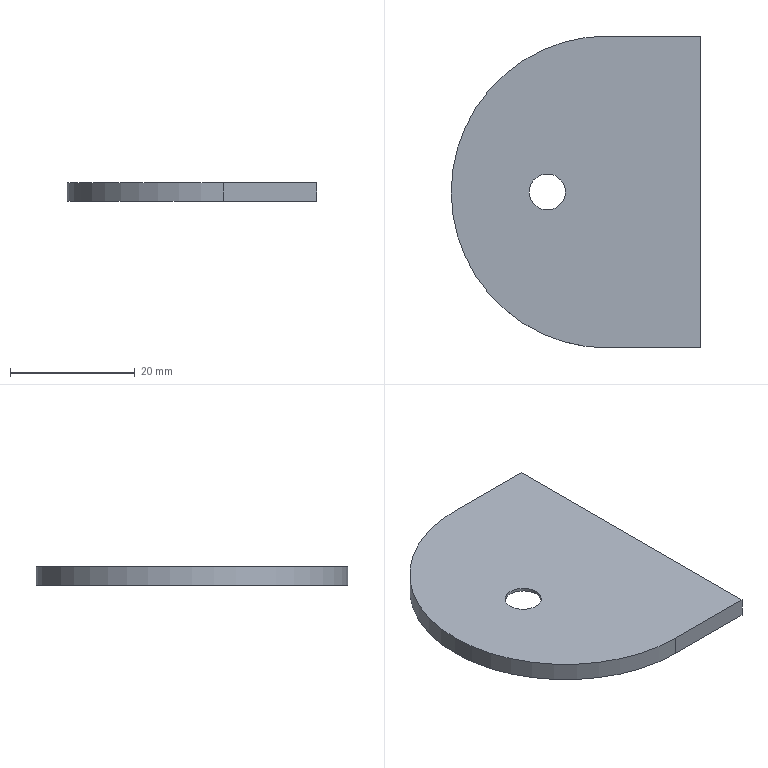Component | NX | HOUSING_COVER | 1 solid | 12 faces | box 40 x 50 x 3 mm | volume 1049 mm3 | plane 9 | cylinder 3 | commonest cylinder face diameters 50 x1 49 x1 5.8 x1
STEP:
#1=CARTESIAN_POINT('',(0.,0.,0.));
#2=DIRECTION('',(0.,0.,1.));
#3=DIRECTION('',(1.,0.,0.));
#4=AXIS2_PLACEMENT_3D('',#1,#2,#3);
#5=CARTESIAN_POINT('',(40.11,76.025,23.712));
#6=VERTEX_POINT('',#5);
#7=CARTESIAN_POINT('',(40.11,26.025,23.712));
#8=VERTEX_POINT('',#7);
#9=CARTESIAN_POINT('',(40.11,51.025,23.712));
#10=DIRECTION('',(0.,0.,1.));
#11=DIRECTION('',(1.,0.,0.));
#12=AXIS2_PLACEMENT_3D('',#9,#10,#11);
#13=CIRCLE('',#12,25.);
#14=CARTESIAN_POINT('',(40.11,51.025,20.712));
#15=DIRECTION('',(0.,0.,1.));
#16=DIRECTION('',(1.,0.,0.));
#17=AXIS2_PLACEMENT_3D('',#14,#15,#16);
#18=CYLINDRICAL_SURFACE('',#17,25.);
#19=CARTESIAN_POINT('',(0.,3.));
#20=DIRECTION('',(1.,0.));
#21=VECTOR('',#20,1.);
#22=LINE('',#19,#21);
#23=(GEOMETRIC_REPRESENTATION_CONTEXT(2)PARAMETRIC_REPRESENTATION_CONTEXT()REPRESENTATION_CONTEXT('',''));
#24=DEFINITIONAL_REPRESENTATION('',(#22),#23);
#25=PCURVE('',#18,#24);
#26=CARTESIAN_POINT('',(40.11,51.025,23.712));
#27=DIRECTION('',(0.,0.,1.));
#28=DIRECTION('',(1.,0.,0.));
#29=AXIS2_PLACEMENT_3D('',#26,#27,#28);
#30=PLANE('',#29);
#31=CARTESIAN_POINT('',(0.,0.));
#32=DIRECTION('',(1.,0.));
#33=AXIS2_PLACEMENT_2D('',#31,#32);
#34=CIRCLE('',#33,25.);
#35=(GEOMETRIC_REPRESENTATION_CONTEXT(2)PARAMETRIC_REPRESENTATION_CONTEXT()REPRESENTATION_CONTEXT('',''));
#36=DEFINITIONAL_REPRESENTATION('',(#34),#35);
#37=PCURVE('',#30,#36);
#38=SURFACE_CURVE('',#13,(#25,#37),.PCURVE_S1.);
#39=EDGE_CURVE('',#6,#8,#38,.T.);
#40=ORIENTED_EDGE('',*,*,#39,.F.);
#41=CARTESIAN_POINT('',(40.11,76.025,20.712));
#42=VERTEX_POINT('',#41);
#43=CARTESIAN_POINT('',(40.11,76.025,20.712));
#44=DIRECTION('',(0.,0.,1.));
#45=VECTOR('',#44,1.);
#46=LINE('',#43,#45);
#47=CARTESIAN_POINT('',(1.571,0.));
#48=DIRECTION('',(0.,1.));
#49=VECTOR('',#48,1.);
#50=LINE('',#47,#49);
#51=(GEOMETRIC_REPRESENTATION_CONTEXT(2)PARAMETRIC_REPRESENTATION_CONTEXT()REPRESENTATION_CONTEXT('',''));
#52=DEFINITIONAL_REPRESENTATION('',(#50),#51);
#53=PCURVE('',#18,#52);
#54=CARTESIAN_POINT('',(55.11,76.025,20.712));
#55=DIRECTION('',(0.,1.,0.));
#56=DIRECTION('',(0.,0.,1.));
#57=AXIS2_PLACEMENT_3D('',#54,#55,#56);
#58=PLANE('',#57);
#59=CARTESIAN_POINT('',(0.,-15.));
#60=DIRECTION('',(1.,0.));
#61=VECTOR('',#60,1.);
#62=LINE('',#59,#61);
#63=(GEOMETRIC_REPRESENTATION_CONTEXT(2)PARAMETRIC_REPRESENTATION_CONTEXT()REPRESENTATION_CONTEXT('',''));
#64=DEFINITIONAL_REPRESENTATION('',(#62),#63);
#65=PCURVE('',#58,#64);
#66=SURFACE_CURVE('',#46,(#53,#65),.PCURVE_S1.);
#67=EDGE_CURVE('',#42,#6,#66,.T.);
#68=ORIENTED_EDGE('',*,*,#67,.F.);
#69=CARTESIAN_POINT('',(40.11,26.025,20.712));
#70=VERTEX_POINT('',#69);
#71=CARTESIAN_POINT('',(40.11,51.025,20.712));
#72=DIRECTION('',(0.,0.,1.));
#73=DIRECTION('',(1.,0.,0.));
#74=AXIS2_PLACEMENT_3D('',#71,#72,#73);
#75=CIRCLE('',#74,25.);
#76=CARTESIAN_POINT('',(0.,0.));
#77=DIRECTION('',(1.,0.));
#78=VECTOR('',#77,1.);
#79=LINE('',#76,#78);
#80=(GEOMETRIC_REPRESENTATION_CONTEXT(2)PARAMETRIC_REPRESENTATION_CONTEXT()REPRESENTATION_CONTEXT('',''));
#81=DEFINITIONAL_REPRESENTATION('',(#79),#80);
#82=PCURVE('',#18,#81);
#83=CARTESIAN_POINT('',(40.11,51.025,20.712));
#84=DIRECTION('',(0.,0.,1.));
#85=DIRECTION('',(1.,0.,0.));
#86=AXIS2_PLACEMENT_3D('',#83,#84,#85);
#87=PLANE('',#86);
#88=CARTESIAN_POINT('',(0.,0.));
#89=DIRECTION('',(1.,0.));
#90=AXIS2_PLACEMENT_2D('',#88,#89);
#91=CIRCLE('',#90,25.);
#92=(GEOMETRIC_REPRESENTATION_CONTEXT(2)PARAMETRIC_REPRESENTATION_CONTEXT()REPRESENTATION_CONTEXT('',''));
#93=DEFINITIONAL_REPRESENTATION('',(#91),#92);
#94=PCURVE('',#87,#93);
#95=SURFACE_CURVE('',#75,(#82,#94),.PCURVE_S1.);
#96=EDGE_CURVE('',#42,#70,#95,.T.);
#97=ORIENTED_EDGE('',*,*,#96,.T.);
#98=CARTESIAN_POINT('',(40.11,26.025,20.712));
#99=DIRECTION('',(0.,0.,1.));
#100=VECTOR('',#99,1.);
#101=LINE('',#98,#100);
#102=CARTESIAN_POINT('',(4.712,0.));
#103=DIRECTION('',(0.,1.));
#104=VECTOR('',#103,1.);
#105=LINE('',#102,#104);
#106=(GEOMETRIC_REPRESENTATION_CONTEXT(2)PARAMETRIC_REPRESENTATION_CONTEXT()REPRESENTATION_CONTEXT('',''));
#107=DEFINITIONAL_REPRESENTATION('',(#105),#106);
#108=PCURVE('',#18,#107);
#109=CARTESIAN_POINT('',(40.11,26.025,20.712));
#110=DIRECTION('',(0.,-1.,0.));
#111=DIRECTION('',(0.,0.,-1.));
#112=AXIS2_PLACEMENT_3D('',#109,#110,#111);
#113=PLANE('',#112);
#114=CARTESIAN_POINT('',(0.,0.));
#115=DIRECTION('',(-1.,0.));
#116=VECTOR('',#115,1.);
#117=LINE('',#114,#116);
#118=(GEOMETRIC_REPRESENTATION_CONTEXT(2)PARAMETRIC_REPRESENTATION_CONTEXT()REPRESENTATION_CONTEXT('',''));
#119=DEFINITIONAL_REPRESENTATION('',(#117),#118);
#120=PCURVE('',#113,#119);
#121=SURFACE_CURVE('',#101,(#108,#120),.PCURVE_S1.);
#122=EDGE_CURVE('',#70,#8,#121,.T.);
#123=ORIENTED_EDGE('',*,*,#122,.T.);
#124=EDGE_LOOP('',(#40,#68,#97,#123));
#125=FACE_BOUND('',#124,.T.);
#126=ADVANCED_FACE('',(#125),#18,.T.);
#127=CARTESIAN_POINT('',(55.11,26.025,23.712));
#128=VERTEX_POINT('',#127);
#129=CARTESIAN_POINT('',(40.11,26.025,23.712));
#130=DIRECTION('',(1.,0.,0.));
#131=VECTOR('',#130,1.);
#132=LINE('',#129,#131);
#133=CARTESIAN_POINT('',(-3.,0.));
#134=DIRECTION('',(0.,1.));
#135=VECTOR('',#134,1.);
#136=LINE('',#133,#135);
#137=(GEOMETRIC_REPRESENTATION_CONTEXT(2)PARAMETRIC_REPRESENTATION_CONTEXT()REPRESENTATION_CONTEXT('',''));
#138=DEFINITIONAL_REPRESENTATION('',(#136),#137);
#139=PCURVE('',#113,#138);
#140=CARTESIAN_POINT('',(0.,-25.));
#141=DIRECTION('',(1.,0.));
#142=VECTOR('',#141,1.);
#143=LINE('',#140,#142);
#144=(GEOMETRIC_REPRESENTATION_CONTEXT(2)PARAMETRIC_REPRESENTATION_CONTEXT()REPRESENTATION_CONTEXT('',''));
#145=DEFINITIONAL_REPRESENTATION('',(#143),#144);
#146=PCURVE('',#30,#145);
#147=SURFACE_CURVE('',#132,(#139,#146),.PCURVE_S1.);
#148=EDGE_CURVE('',#8,#128,#147,.T.);
#149=ORIENTED_EDGE('',*,*,#148,.F.);
#150=ORIENTED_EDGE('',*,*,#122,.F.);
#151=CARTESIAN_POINT('',(55.11,26.025,20.712));
#152=VERTEX_POINT('',#151);
#153=CARTESIAN_POINT('',(40.11,26.025,20.712));
#154=DIRECTION('',(1.,0.,0.));
#155=VECTOR('',#154,1.);
#156=LINE('',#153,#155);
#157=CARTESIAN_POINT('',(0.,0.));
#158=DIRECTION('',(0.,1.));
#159=VECTOR('',#158,1.);
#160=LINE('',#157,#159);
#161=(GEOMETRIC_REPRESENTATION_CONTEXT(2)PARAMETRIC_REPRESENTATION_CONTEXT()REPRESENTATION_CONTEXT('',''));
#162=DEFINITIONAL_REPRESENTATION('',(#160),#161);
#163=PCURVE('',#113,#162);
#164=CARTESIAN_POINT('',(0.,-25.));
#165=DIRECTION('',(1.,0.));
#166=VECTOR('',#165,1.);
#167=LINE('',#164,#166);
#168=(GEOMETRIC_REPRESENTATION_CONTEXT(2)PARAMETRIC_REPRESENTATION_CONTEXT()REPRESENTATION_CONTEXT('',''));
#169=DEFINITIONAL_REPRESENTATION('',(#167),#168);
#170=PCURVE('',#87,#169);
#171=SURFACE_CURVE('',#156,(#163,#170),.PCURVE_S1.);
#172=EDGE_CURVE('',#70,#152,#171,.T.);
#173=ORIENTED_EDGE('',*,*,#172,.T.);
#174=CARTESIAN_POINT('',(55.11,26.025,20.712));
#175=DIRECTION('',(0.,0.,1.));
#176=VECTOR('',#175,1.);
#177=LINE('',#174,#176);
#178=CARTESIAN_POINT('',(0.,15.));
#179=DIRECTION('',(-1.,0.));
#180=VECTOR('',#179,1.);
#181=LINE('',#178,#180);
#182=(GEOMETRIC_REPRESENTATION_CONTEXT(2)PARAMETRIC_REPRESENTATION_CONTEXT()REPRESENTATION_CONTEXT('',''));
#183=DEFINITIONAL_REPRESENTATION('',(#181),#182);
#184=PCURVE('',#113,#183);
#185=CARTESIAN_POINT('',(55.11,26.025,20.712));
#186=DIRECTION('',(1.,0.,0.));
#187=DIRECTION('',(-0.,1.,0.));
#188=AXIS2_PLACEMENT_3D('',#185,#186,#187);
#189=PLANE('',#188);
#190=CARTESIAN_POINT('',(0.,0.));
#191=DIRECTION('',(0.,1.));
#192=VECTOR('',#191,1.);
#193=LINE('',#190,#192);
#194=(GEOMETRIC_REPRESENTATION_CONTEXT(2)PARAMETRIC_REPRESENTATION_CONTEXT()REPRESENTATION_CONTEXT('',''));
#195=DEFINITIONAL_REPRESENTATION('',(#193),#194);
#196=PCURVE('',#189,#195);
#197=SURFACE_CURVE('',#177,(#184,#196),.PCURVE_S1.);
#198=EDGE_CURVE('',#152,#128,#197,.T.);
#199=ORIENTED_EDGE('',*,*,#198,.T.);
#200=EDGE_LOOP('',(#149,#150,#173,#199));
#201=FACE_BOUND('',#200,.T.);
#202=ADVANCED_FACE('',(#201),#113,.T.);
#203=CARTESIAN_POINT('',(55.11,76.025,23.712));
#204=VERTEX_POINT('',#203);
#205=CARTESIAN_POINT('',(55.11,26.025,23.712));
#206=DIRECTION('',(-0.,1.,0.));
#207=VECTOR('',#206,1.);
#208=LINE('',#205,#207);
#209=CARTESIAN_POINT('',(0.,3.));
#210=DIRECTION('',(1.,0.));
#211=VECTOR('',#210,1.);
#212=LINE('',#209,#211);
#213=(GEOMETRIC_REPRESENTATION_CONTEXT(2)PARAMETRIC_REPRESENTATION_CONTEXT()REPRESENTATION_CONTEXT('',''));
#214=DEFINITIONAL_REPRESENTATION('',(#212),#213);
#215=PCURVE('',#189,#214);
#216=CARTESIAN_POINT('',(15.,-25.));
#217=DIRECTION('',(-0.,1.));
#218=VECTOR('',#217,1.);
#219=LINE('',#216,#218);
#220=(GEOMETRIC_REPRESENTATION_CONTEXT(2)PARAMETRIC_REPRESENTATION_CONTEXT()REPRESENTATION_CONTEXT('',''));
#221=DEFINITIONAL_REPRESENTATION('',(#219),#220);
#222=PCURVE('',#30,#221);
#223=SURFACE_CURVE('',#208,(#215,#222),.PCURVE_S1.);
#224=EDGE_CURVE('',#128,#204,#223,.T.);
#225=ORIENTED_EDGE('',*,*,#224,.F.);
#226=ORIENTED_EDGE('',*,*,#198,.F.);
#227=CARTESIAN_POINT('',(55.11,76.025,20.712));
#228=VERTEX_POINT('',#227);
#229=CARTESIAN_POINT('',(55.11,26.025,20.712));
#230=DIRECTION('',(-0.,1.,0.));
#231=VECTOR('',#230,1.);
#232=LINE('',#229,#231);
#233=CARTESIAN_POINT('',(0.,0.));
#234=DIRECTION('',(1.,0.));
#235=VECTOR('',#234,1.);
#236=LINE('',#233,#235);
#237=(GEOMETRIC_REPRESENTATION_CONTEXT(2)PARAMETRIC_REPRESENTATION_CONTEXT()REPRESENTATION_CONTEXT('',''));
#238=DEFINITIONAL_REPRESENTATION('',(#236),#237);
#239=PCURVE('',#189,#238);
#240=CARTESIAN_POINT('',(15.,-25.));
#241=DIRECTION('',(-0.,1.));
#242=VECTOR('',#241,1.);
#243=LINE('',#240,#242);
#244=(GEOMETRIC_REPRESENTATION_CONTEXT(2)PARAMETRIC_REPRESENTATION_CONTEXT()REPRESENTATION_CONTEXT('',''));
#245=DEFINITIONAL_REPRESENTATION('',(#243),#244);
#246=PCURVE('',#87,#245);
#247=SURFACE_CURVE('',#232,(#239,#246),.PCURVE_S1.);
#248=EDGE_CURVE('',#152,#228,#247,.T.);
#249=ORIENTED_EDGE('',*,*,#248,.T.);
#250=CARTESIAN_POINT('',(55.11,76.025,20.712));
#251=DIRECTION('',(0.,0.,1.));
#252=VECTOR('',#251,1.);
#253=LINE('',#250,#252);
#254=CARTESIAN_POINT('',(50.,0.));
#255=DIRECTION('',(0.,1.));
#256=VECTOR('',#255,1.);
#257=LINE('',#254,#256);
#258=(GEOMETRIC_REPRESENTATION_CONTEXT(2)PARAMETRIC_REPRESENTATION_CONTEXT()REPRESENTATION_CONTEXT('',''));
#259=DEFINITIONAL_REPRESENTATION('',(#257),#258);
#260=PCURVE('',#189,#259);
#261=CARTESIAN_POINT('',(0.,0.));
#262=DIRECTION('',(1.,0.));
#263=VECTOR('',#262,1.);
#264=LINE('',#261,#263);
#265=(GEOMETRIC_REPRESENTATION_CONTEXT(2)PARAMETRIC_REPRESENTATION_CONTEXT()REPRESENTATION_CONTEXT('',''));
#266=DEFINITIONAL_REPRESENTATION('',(#264),#265);
#267=PCURVE('',#58,#266);
#268=SURFACE_CURVE('',#253,(#260,#267),.PCURVE_S1.);
#269=EDGE_CURVE('',#228,#204,#268,.T.);
#270=ORIENTED_EDGE('',*,*,#269,.T.);
#271=EDGE_LOOP('',(#225,#226,#249,#270));
#272=FACE_BOUND('',#271,.T.);
#273=ADVANCED_FACE('',(#272),#189,.T.);
#274=CARTESIAN_POINT('',(55.11,76.025,23.712));
#275=DIRECTION('',(-1.,0.,0.));
#276=VECTOR('',#275,1.);
#277=LINE('',#274,#276);
#278=CARTESIAN_POINT('',(3.,0.));
#279=DIRECTION('',(0.,-1.));
#280=VECTOR('',#279,1.);
#281=LINE('',#278,#280);
#282=(GEOMETRIC_REPRESENTATION_CONTEXT(2)PARAMETRIC_REPRESENTATION_CONTEXT()REPRESENTATION_CONTEXT('',''));
#283=DEFINITIONAL_REPRESENTATION('',(#281),#282);
#284=PCURVE('',#58,#283);
#285=CARTESIAN_POINT('',(15.,25.));
#286=DIRECTION('',(-1.,0.));
#287=VECTOR('',#286,1.);
#288=LINE('',#285,#287);
#289=(GEOMETRIC_REPRESENTATION_CONTEXT(2)PARAMETRIC_REPRESENTATION_CONTEXT()REPRESENTATION_CONTEXT('',''));
#290=DEFINITIONAL_REPRESENTATION('',(#288),#289);
#291=PCURVE('',#30,#290);
#292=SURFACE_CURVE('',#277,(#284,#291),.PCURVE_S1.);
#293=EDGE_CURVE('',#204,#6,#292,.T.);
#294=ORIENTED_EDGE('',*,*,#293,.F.);
#295=ORIENTED_EDGE('',*,*,#269,.F.);
#296=CARTESIAN_POINT('',(55.11,76.025,20.712));
#297=DIRECTION('',(-1.,0.,0.));
#298=VECTOR('',#297,1.);
#299=LINE('',#296,#298);
#300=CARTESIAN_POINT('',(0.,0.));
#301=DIRECTION('',(0.,-1.));
#302=VECTOR('',#301,1.);
#303=LINE('',#300,#302);
#304=(GEOMETRIC_REPRESENTATION_CONTEXT(2)PARAMETRIC_REPRESENTATION_CONTEXT()REPRESENTATION_CONTEXT('',''));
#305=DEFINITIONAL_REPRESENTATION('',(#303),#304);
#306=PCURVE('',#58,#305);
#307=CARTESIAN_POINT('',(15.,25.));
#308=DIRECTION('',(-1.,0.));
#309=VECTOR('',#308,1.);
#310=LINE('',#307,#309);
#311=(GEOMETRIC_REPRESENTATION_CONTEXT(2)PARAMETRIC_REPRESENTATION_CONTEXT()REPRESENTATION_CONTEXT('',''));
#312=DEFINITIONAL_REPRESENTATION('',(#310),#311);
#313=PCURVE('',#87,#312);
#314=SURFACE_CURVE('',#299,(#306,#313),.PCURVE_S1.);
#315=EDGE_CURVE('',#228,#42,#314,.T.);
#316=ORIENTED_EDGE('',*,*,#315,.T.);
#317=ORIENTED_EDGE('',*,*,#67,.T.);
#318=EDGE_LOOP('',(#294,#295,#316,#317));
#319=FACE_BOUND('',#318,.T.);
#320=ADVANCED_FACE('',(#319),#58,.T.);
#321=CARTESIAN_POINT('',(54.61,75.525,20.712));
#322=VERTEX_POINT('',#321);
#323=CARTESIAN_POINT('',(40.11,75.525,20.712));
#324=VERTEX_POINT('',#323);
#325=CARTESIAN_POINT('',(40.11,75.525,20.712));
#326=DIRECTION('',(-1.,0.,0.));
#327=VECTOR('',#326,1.);
#328=LINE('',#325,#327);
#329=CARTESIAN_POINT('',(0.,24.5));
#330=DIRECTION('',(-1.,0.));
#331=VECTOR('',#330,1.);
#332=LINE('',#329,#331);
#333=(GEOMETRIC_REPRESENTATION_CONTEXT(2)PARAMETRIC_REPRESENTATION_CONTEXT()REPRESENTATION_CONTEXT('',''));
#334=DEFINITIONAL_REPRESENTATION('',(#332),#333);
#335=PCURVE('',#87,#334);
#336=CARTESIAN_POINT('',(55.11,75.525,20.712));
#337=DIRECTION('',(0.,1.,0.));
#338=DIRECTION('',(0.,0.,1.));
#339=AXIS2_PLACEMENT_3D('',#336,#337,#338);
#340=PLANE('',#339);
#341=CARTESIAN_POINT('',(0.,-15.));
#342=DIRECTION('',(0.,-1.));
#343=VECTOR('',#342,1.);
#344=LINE('',#341,#343);
#345=(GEOMETRIC_REPRESENTATION_CONTEXT(2)PARAMETRIC_REPRESENTATION_CONTEXT()REPRESENTATION_CONTEXT('',''));
#346=DEFINITIONAL_REPRESENTATION('',(#344),#345);
#347=PCURVE('',#340,#346);
#348=SURFACE_CURVE('',#328,(#335,#347),.PCURVE_S1.);
#349=EDGE_CURVE('',#322,#324,#348,.T.);
#350=ORIENTED_EDGE('',*,*,#349,.T.);
#351=CARTESIAN_POINT('',(40.11,26.525,20.712));
#352=VERTEX_POINT('',#351);
#353=CARTESIAN_POINT('',(40.11,51.025,20.712));
#354=DIRECTION('',(0.,0.,1.));
#355=DIRECTION('',(1.,0.,0.));
#356=AXIS2_PLACEMENT_3D('',#353,#354,#355);
#357=CIRCLE('',#356,24.5);
#358=CARTESIAN_POINT('',(0.,0.));
#359=DIRECTION('',(1.,0.));
#360=AXIS2_PLACEMENT_2D('',#358,#359);
#361=CIRCLE('',#360,24.5);
#362=(GEOMETRIC_REPRESENTATION_CONTEXT(2)PARAMETRIC_REPRESENTATION_CONTEXT()REPRESENTATION_CONTEXT('',''));
#363=DEFINITIONAL_REPRESENTATION('',(#361),#362);
#364=PCURVE('',#87,#363);
#365=CARTESIAN_POINT('',(40.11,51.025,20.712));
#366=DIRECTION('',(0.,0.,1.));
#367=DIRECTION('',(1.,0.,0.));
#368=AXIS2_PLACEMENT_3D('',#365,#366,#367);
#369=CYLINDRICAL_SURFACE('',#368,24.5);
#370=CARTESIAN_POINT('',(0.,0.));
#371=DIRECTION('',(1.,0.));
#372=VECTOR('',#371,1.);
#373=LINE('',#370,#372);
#374=(GEOMETRIC_REPRESENTATION_CONTEXT(2)PARAMETRIC_REPRESENTATION_CONTEXT()REPRESENTATION_CONTEXT('',''));
#375=DEFINITIONAL_REPRESENTATION('',(#373),#374);
#376=PCURVE('',#369,#375);
#377=SURFACE_CURVE('',#357,(#364,#376),.PCURVE_S1.);
#378=EDGE_CURVE('',#324,#352,#377,.T.);
#379=ORIENTED_EDGE('',*,*,#378,.T.);
#380=CARTESIAN_POINT('',(54.61,26.525,20.712));
#381=VERTEX_POINT('',#380);
#382=CARTESIAN_POINT('',(40.11,26.525,20.712));
#383=DIRECTION('',(1.,0.,0.));
#384=VECTOR('',#383,1.);
#385=LINE('',#382,#384);
#386=CARTESIAN_POINT('',(0.,-24.5));
#387=DIRECTION('',(1.,0.));
#388=VECTOR('',#387,1.);
#389=LINE('',#386,#388);
#390=(GEOMETRIC_REPRESENTATION_CONTEXT(2)PARAMETRIC_REPRESENTATION_CONTEXT()REPRESENTATION_CONTEXT('',''));
#391=DEFINITIONAL_REPRESENTATION('',(#389),#390);
#392=PCURVE('',#87,#391);
#393=CARTESIAN_POINT('',(40.11,26.525,20.712));
#394=DIRECTION('',(0.,-1.,0.));
#395=DIRECTION('',(0.,0.,-1.));
#396=AXIS2_PLACEMENT_3D('',#393,#394,#395);
#397=PLANE('',#396);
#398=CARTESIAN_POINT('',(0.,0.));
#399=DIRECTION('',(0.,1.));
#400=VECTOR('',#399,1.);
#401=LINE('',#398,#400);
#402=(GEOMETRIC_REPRESENTATION_CONTEXT(2)PARAMETRIC_REPRESENTATION_CONTEXT()REPRESENTATION_CONTEXT('',''));
#403=DEFINITIONAL_REPRESENTATION('',(#401),#402);
#404=PCURVE('',#397,#403);
#405=SURFACE_CURVE('',#385,(#392,#404),.PCURVE_S1.);
#406=EDGE_CURVE('',#352,#381,#405,.T.);
#407=ORIENTED_EDGE('',*,*,#406,.T.);
#408=CARTESIAN_POINT('',(54.61,51.025,20.712));
#409=DIRECTION('',(-0.,1.,0.));
#410=VECTOR('',#409,1.);
#411=LINE('',#408,#410);
#412=CARTESIAN_POINT('',(14.5,0.));
#413=DIRECTION('',(-0.,1.));
#414=VECTOR('',#413,1.);
#415=LINE('',#412,#414);
#416=(GEOMETRIC_REPRESENTATION_CONTEXT(2)PARAMETRIC_REPRESENTATION_CONTEXT()REPRESENTATION_CONTEXT('',''));
#417=DEFINITIONAL_REPRESENTATION('',(#415),#416);
#418=PCURVE('',#87,#417);
#419=CARTESIAN_POINT('',(54.61,26.025,20.712));
#420=DIRECTION('',(1.,0.,0.));
#421=DIRECTION('',(-0.,1.,0.));
#422=AXIS2_PLACEMENT_3D('',#419,#420,#421);
#423=PLANE('',#422);
#424=CARTESIAN_POINT('',(25.,0.));
#425=DIRECTION('',(1.,0.));
#426=VECTOR('',#425,1.);
#427=LINE('',#424,#426);
#428=(GEOMETRIC_REPRESENTATION_CONTEXT(2)PARAMETRIC_REPRESENTATION_CONTEXT()REPRESENTATION_CONTEXT('',''));
#429=DEFINITIONAL_REPRESENTATION('',(#427),#428);
#430=PCURVE('',#423,#429);
#431=SURFACE_CURVE('',#411,(#418,#430),.PCURVE_S1.);
#432=EDGE_CURVE('',#381,#322,#431,.T.);
#433=ORIENTED_EDGE('',*,*,#432,.T.);
#434=EDGE_LOOP('',(#350,#379,#407,#433));
#435=FACE_BOUND('',#434,.T.);
#436=ORIENTED_EDGE('',*,*,#96,.F.);
#437=ORIENTED_EDGE('',*,*,#315,.F.);
#438=ORIENTED_EDGE('',*,*,#248,.F.);
#439=ORIENTED_EDGE('',*,*,#172,.F.);
#440=EDGE_LOOP('',(#436,#437,#438,#439));
#441=FACE_BOUND('',#440,.T.);
#442=ADVANCED_FACE('',(#435,#441),#87,.F.);
#443=CARTESIAN_POINT('',(33.41,51.025,23.712));
#444=VERTEX_POINT('',#443);
#445=CARTESIAN_POINT('',(30.51,51.025,23.712));
#446=DIRECTION('',(0.,0.,1.));
#447=DIRECTION('',(1.,0.,0.));
#448=AXIS2_PLACEMENT_3D('',#445,#446,#447);
#449=CIRCLE('',#448,2.9);
#450=CARTESIAN_POINT('',(-9.6,0.));
#451=DIRECTION('',(1.,0.));
#452=AXIS2_PLACEMENT_2D('',#450,#451);
#453=CIRCLE('',#452,2.9);
#454=(GEOMETRIC_REPRESENTATION_CONTEXT(2)PARAMETRIC_REPRESENTATION_CONTEXT()REPRESENTATION_CONTEXT('',''));
#455=DEFINITIONAL_REPRESENTATION('',(#453),#454);
#456=PCURVE('',#30,#455);
#457=CARTESIAN_POINT('',(30.51,51.025,23.712));
#458=DIRECTION('',(0.,0.,-1.));
#459=DIRECTION('',(-1.,0.,0.));
#460=AXIS2_PLACEMENT_3D('',#457,#458,#459);
#461=CYLINDRICAL_SURFACE('',#460,2.9);
#462=CARTESIAN_POINT('',(9.425,0.));
#463=DIRECTION('',(-1.,0.));
#464=VECTOR('',#463,1.);
#465=LINE('',#462,#464);
#466=(GEOMETRIC_REPRESENTATION_CONTEXT(2)PARAMETRIC_REPRESENTATION_CONTEXT()REPRESENTATION_CONTEXT('',''));
#467=DEFINITIONAL_REPRESENTATION('',(#465),#466);
#468=PCURVE('',#461,#467);
#469=SURFACE_CURVE('',#449,(#456,#468),.PCURVE_S1.);
#470=EDGE_CURVE('',#444,#444,#469,.T.);
#471=ORIENTED_EDGE('',*,*,#470,.F.);
#472=EDGE_LOOP('',(#471));
#473=FACE_BOUND('',#472,.T.);
#474=ORIENTED_EDGE('',*,*,#39,.T.);
#475=ORIENTED_EDGE('',*,*,#148,.T.);
#476=ORIENTED_EDGE('',*,*,#224,.T.);
#477=ORIENTED_EDGE('',*,*,#293,.T.);
#478=EDGE_LOOP('',(#474,#475,#476,#477));
#479=FACE_BOUND('',#478,.T.);
#480=ADVANCED_FACE('',(#473,#479),#30,.T.);
#481=CARTESIAN_POINT('',(40.11,75.525,23.212));
#482=VERTEX_POINT('',#481);
#483=CARTESIAN_POINT('',(40.11,75.525,20.712));
#484=DIRECTION('',(0.,0.,1.));
#485=VECTOR('',#484,1.);
#486=LINE('',#483,#485);
#487=CARTESIAN_POINT('',(1.571,0.));
#488=DIRECTION('',(0.,1.));
#489=VECTOR('',#488,1.);
#490=LINE('',#487,#489);
#491=(GEOMETRIC_REPRESENTATION_CONTEXT(2)PARAMETRIC_REPRESENTATION_CONTEXT()REPRESENTATION_CONTEXT('',''));
#492=DEFINITIONAL_REPRESENTATION('',(#490),#491);
#493=PCURVE('',#369,#492);
#494=CARTESIAN_POINT('',(0.,-15.));
#495=DIRECTION('',(1.,0.));
#496=VECTOR('',#495,1.);
#497=LINE('',#494,#496);
#498=(GEOMETRIC_REPRESENTATION_CONTEXT(2)PARAMETRIC_REPRESENTATION_CONTEXT()REPRESENTATION_CONTEXT('',''));
#499=DEFINITIONAL_REPRESENTATION('',(#497),#498);
#500=PCURVE('',#340,#499);
#501=SURFACE_CURVE('',#486,(#493,#500),.PCURVE_S1.);
#502=EDGE_CURVE('',#324,#482,#501,.T.);
#503=ORIENTED_EDGE('',*,*,#502,.F.);
#504=ORIENTED_EDGE('',*,*,#378,.T.);
#505=CARTESIAN_POINT('',(40.11,26.525,23.212));
#506=VERTEX_POINT('',#505);
#507=CARTESIAN_POINT('',(40.11,26.525,20.712));
#508=DIRECTION('',(0.,0.,1.));
#509=VECTOR('',#508,1.);
#510=LINE('',#507,#509);
#511=CARTESIAN_POINT('',(4.712,0.));
#512=DIRECTION('',(0.,1.));
#513=VECTOR('',#512,1.);
#514=LINE('',#511,#513);
#515=(GEOMETRIC_REPRESENTATION_CONTEXT(2)PARAMETRIC_REPRESENTATION_CONTEXT()REPRESENTATION_CONTEXT('',''));
#516=DEFINITIONAL_REPRESENTATION('',(#514),#515);
#517=PCURVE('',#369,#516);
#518=CARTESIAN_POINT('',(0.,0.));
#519=DIRECTION('',(-1.,0.));
#520=VECTOR('',#519,1.);
#521=LINE('',#518,#520);
#522=(GEOMETRIC_REPRESENTATION_CONTEXT(2)PARAMETRIC_REPRESENTATION_CONTEXT()REPRESENTATION_CONTEXT('',''));
#523=DEFINITIONAL_REPRESENTATION('',(#521),#522);
#524=PCURVE('',#397,#523);
#525=SURFACE_CURVE('',#510,(#517,#524),.PCURVE_S1.);
#526=EDGE_CURVE('',#352,#506,#525,.T.);
#527=ORIENTED_EDGE('',*,*,#526,.T.);
#528=CARTESIAN_POINT('',(40.11,51.025,23.212));
#529=DIRECTION('',(0.,0.,1.));
#530=DIRECTION('',(1.,0.,0.));
#531=AXIS2_PLACEMENT_3D('',#528,#529,#530);
#532=CIRCLE('',#531,24.5);
#533=CARTESIAN_POINT('',(0.,2.5));
#534=DIRECTION('',(1.,0.));
#535=VECTOR('',#534,1.);
#536=LINE('',#533,#535);
#537=(GEOMETRIC_REPRESENTATION_CONTEXT(2)PARAMETRIC_REPRESENTATION_CONTEXT()REPRESENTATION_CONTEXT('',''));
#538=DEFINITIONAL_REPRESENTATION('',(#536),#537);
#539=PCURVE('',#369,#538);
#540=CARTESIAN_POINT('',(40.11,51.025,23.212));
#541=DIRECTION('',(0.,0.,1.));
#542=DIRECTION('',(1.,0.,0.));
#543=AXIS2_PLACEMENT_3D('',#540,#541,#542);
#544=PLANE('',#543);
#545=CARTESIAN_POINT('',(0.,0.));
#546=DIRECTION('',(1.,0.));
#547=AXIS2_PLACEMENT_2D('',#545,#546);
#548=CIRCLE('',#547,24.5);
#549=(GEOMETRIC_REPRESENTATION_CONTEXT(2)PARAMETRIC_REPRESENTATION_CONTEXT()REPRESENTATION_CONTEXT('',''));
#550=DEFINITIONAL_REPRESENTATION('',(#548),#549);
#551=PCURVE('',#544,#550);
#552=SURFACE_CURVE('',#532,(#539,#551),.PCURVE_S1.);
#553=EDGE_CURVE('',#482,#506,#552,.T.);
#554=ORIENTED_EDGE('',*,*,#553,.F.);
#555=EDGE_LOOP('',(#503,#504,#527,#554));
#556=FACE_BOUND('',#555,.F.);
#557=ADVANCED_FACE('',(#556),#369,.F.);
#558=CARTESIAN_POINT('',(54.61,26.525,23.212));
#559=VERTEX_POINT('',#558);
#560=CARTESIAN_POINT('',(40.11,26.525,23.212));
#561=DIRECTION('',(1.,0.,0.));
#562=VECTOR('',#561,1.);
#563=LINE('',#560,#562);
#564=CARTESIAN_POINT('',(-2.5,0.));
#565=DIRECTION('',(0.,1.));
#566=VECTOR('',#565,1.);
#567=LINE('',#564,#566);
#568=(GEOMETRIC_REPRESENTATION_CONTEXT(2)PARAMETRIC_REPRESENTATION_CONTEXT()REPRESENTATION_CONTEXT('',''));
#569=DEFINITIONAL_REPRESENTATION('',(#567),#568);
#570=PCURVE('',#397,#569);
#571=CARTESIAN_POINT('',(0.,-24.5));
#572=DIRECTION('',(1.,0.));
#573=VECTOR('',#572,1.);
#574=LINE('',#571,#573);
#575=(GEOMETRIC_REPRESENTATION_CONTEXT(2)PARAMETRIC_REPRESENTATION_CONTEXT()REPRESENTATION_CONTEXT('',''));
#576=DEFINITIONAL_REPRESENTATION('',(#574),#575);
#577=PCURVE('',#544,#576);
#578=SURFACE_CURVE('',#563,(#570,#577),.PCURVE_S1.);
#579=EDGE_CURVE('',#506,#559,#578,.T.);
#580=ORIENTED_EDGE('',*,*,#579,.T.);
#581=CARTESIAN_POINT('',(54.61,26.525,20.712));
#582=DIRECTION('',(0.,0.,1.));
#583=VECTOR('',#582,1.);
#584=LINE('',#581,#583);
#585=CARTESIAN_POINT('',(0.,14.5));
#586=DIRECTION('',(-1.,0.));
#587=VECTOR('',#586,1.);
#588=LINE('',#585,#587);
#589=(GEOMETRIC_REPRESENTATION_CONTEXT(2)PARAMETRIC_REPRESENTATION_CONTEXT()REPRESENTATION_CONTEXT('',''));
#590=DEFINITIONAL_REPRESENTATION('',(#588),#589);
#591=PCURVE('',#397,#590);
#592=CARTESIAN_POINT('',(0.5,0.));
#593=DIRECTION('',(0.,1.));
#594=VECTOR('',#593,1.);
#595=LINE('',#592,#594);
#596=(GEOMETRIC_REPRESENTATION_CONTEXT(2)PARAMETRIC_REPRESENTATION_CONTEXT()REPRESENTATION_CONTEXT('',''));
#597=DEFINITIONAL_REPRESENTATION('',(#595),#596);
#598=PCURVE('',#423,#597);
#599=SURFACE_CURVE('',#584,(#591,#598),.PCURVE_S1.);
#600=EDGE_CURVE('',#381,#559,#599,.T.);
#601=ORIENTED_EDGE('',*,*,#600,.F.);
#602=ORIENTED_EDGE('',*,*,#406,.F.);
#603=ORIENTED_EDGE('',*,*,#526,.T.);
#604=EDGE_LOOP('',(#580,#601,#602,#603));
#605=FACE_BOUND('',#604,.T.);
#606=ADVANCED_FACE('',(#605),#397,.F.);
#607=CARTESIAN_POINT('',(54.61,75.525,23.212));
#608=VERTEX_POINT('',#607);
#609=CARTESIAN_POINT('',(54.61,51.025,23.212));
#610=DIRECTION('',(-0.,1.,0.));
#611=VECTOR('',#610,1.);
#612=LINE('',#609,#611);
#613=CARTESIAN_POINT('',(25.,2.5));
#614=DIRECTION('',(1.,0.));
#615=VECTOR('',#614,1.);
#616=LINE('',#613,#615);
#617=(GEOMETRIC_REPRESENTATION_CONTEXT(2)PARAMETRIC_REPRESENTATION_CONTEXT()REPRESENTATION_CONTEXT('',''));
#618=DEFINITIONAL_REPRESENTATION('',(#616),#617);
#619=PCURVE('',#423,#618);
#620=CARTESIAN_POINT('',(14.5,0.));
#621=DIRECTION('',(-0.,1.));
#622=VECTOR('',#621,1.);
#623=LINE('',#620,#622);
#624=(GEOMETRIC_REPRESENTATION_CONTEXT(2)PARAMETRIC_REPRESENTATION_CONTEXT()REPRESENTATION_CONTEXT('',''));
#625=DEFINITIONAL_REPRESENTATION('',(#623),#624);
#626=PCURVE('',#544,#625);
#627=SURFACE_CURVE('',#612,(#619,#626),.PCURVE_S1.);
#628=EDGE_CURVE('',#559,#608,#627,.T.);
#629=ORIENTED_EDGE('',*,*,#628,.T.);
#630=CARTESIAN_POINT('',(54.61,75.525,20.712));
#631=DIRECTION('',(0.,0.,1.));
#632=VECTOR('',#631,1.);
#633=LINE('',#630,#632);
#634=CARTESIAN_POINT('',(49.5,0.));
#635=DIRECTION('',(0.,1.));
#636=VECTOR('',#635,1.);
#637=LINE('',#634,#636);
#638=(GEOMETRIC_REPRESENTATION_CONTEXT(2)PARAMETRIC_REPRESENTATION_CONTEXT()REPRESENTATION_CONTEXT('',''));
#639=DEFINITIONAL_REPRESENTATION('',(#637),#638);
#640=PCURVE('',#423,#639);
#641=CARTESIAN_POINT('',(0.,-0.5));
#642=DIRECTION('',(1.,0.));
#643=VECTOR('',#642,1.);
#644=LINE('',#641,#643);
#645=(GEOMETRIC_REPRESENTATION_CONTEXT(2)PARAMETRIC_REPRESENTATION_CONTEXT()REPRESENTATION_CONTEXT('',''));
#646=DEFINITIONAL_REPRESENTATION('',(#644),#645);
#647=PCURVE('',#340,#646);
#648=SURFACE_CURVE('',#633,(#640,#647),.PCURVE_S1.);
#649=EDGE_CURVE('',#322,#608,#648,.T.);
#650=ORIENTED_EDGE('',*,*,#649,.F.);
#651=ORIENTED_EDGE('',*,*,#432,.F.);
#652=ORIENTED_EDGE('',*,*,#600,.T.);
#653=EDGE_LOOP('',(#629,#650,#651,#652));
#654=FACE_BOUND('',#653,.T.);
#655=ADVANCED_FACE('',(#654),#423,.F.);
#656=CARTESIAN_POINT('',(40.11,75.525,23.212));
#657=DIRECTION('',(-1.,0.,0.));
#658=VECTOR('',#657,1.);
#659=LINE('',#656,#658);
#660=CARTESIAN_POINT('',(2.5,-15.));
#661=DIRECTION('',(0.,-1.));
#662=VECTOR('',#661,1.);
#663=LINE('',#660,#662);
#664=(GEOMETRIC_REPRESENTATION_CONTEXT(2)PARAMETRIC_REPRESENTATION_CONTEXT()REPRESENTATION_CONTEXT('',''));
#665=DEFINITIONAL_REPRESENTATION('',(#663),#664);
#666=PCURVE('',#340,#665);
#667=CARTESIAN_POINT('',(0.,24.5));
#668=DIRECTION('',(-1.,0.));
#669=VECTOR('',#668,1.);
#670=LINE('',#667,#669);
#671=(GEOMETRIC_REPRESENTATION_CONTEXT(2)PARAMETRIC_REPRESENTATION_CONTEXT()REPRESENTATION_CONTEXT('',''));
#672=DEFINITIONAL_REPRESENTATION('',(#670),#671);
#673=PCURVE('',#544,#672);
#674=SURFACE_CURVE('',#659,(#666,#673),.PCURVE_S1.);
#675=EDGE_CURVE('',#608,#482,#674,.T.);
#676=ORIENTED_EDGE('',*,*,#675,.T.);
#677=ORIENTED_EDGE('',*,*,#502,.F.);
#678=ORIENTED_EDGE('',*,*,#349,.F.);
#679=ORIENTED_EDGE('',*,*,#649,.T.);
#680=EDGE_LOOP('',(#676,#677,#678,#679));
#681=FACE_BOUND('',#680,.T.);
#682=ADVANCED_FACE('',(#681),#340,.F.);
#683=CARTESIAN_POINT('',(33.41,51.025,23.212));
#684=VERTEX_POINT('',#683);
#685=CARTESIAN_POINT('',(30.51,51.025,23.212));
#686=DIRECTION('',(0.,0.,-1.));
#687=DIRECTION('',(1.,0.,0.));
#688=AXIS2_PLACEMENT_3D('',#685,#686,#687);
#689=CIRCLE('',#688,2.9);
#690=CARTESIAN_POINT('',(-6.7,0.));
#691=CARTESIAN_POINT('',(-6.7,-5.023));
#692=CARTESIAN_POINT('',(-11.05,-2.511));
#693=CARTESIAN_POINT('',(-15.4,-0.));
#694=CARTESIAN_POINT('',(-11.05,2.511));
#695=CARTESIAN_POINT('',(-6.7,5.023));
#696=CARTESIAN_POINT('',(-6.7,0.));
#697=(BOUNDED_CURVE()B_SPLINE_CURVE(2,(#690,#691,#692,#693,#694,#695,#696),.UNSPECIFIED.,.T.,.F.)B_SPLINE_CURVE_WITH_KNOTS((1,2,2,2,2,1),(-2.094,0.,2.094,4.189,6.283,8.378),.UNSPECIFIED.)CURVE()GEOMETRIC_REPRESENTATION_ITEM()RATIONAL_B_SPLINE_CURVE((1.,0.5,1.,0.5,1.,0.5,1.))REPRESENTATION_ITEM(''));
#698=(GEOMETRIC_REPRESENTATION_CONTEXT(2)PARAMETRIC_REPRESENTATION_CONTEXT()REPRESENTATION_CONTEXT('',''));
#699=DEFINITIONAL_REPRESENTATION('',(#697),#698);
#700=PCURVE('',#544,#699);
#701=CARTESIAN_POINT('',(3.142,0.5));
#702=DIRECTION('',(1.,0.));
#703=VECTOR('',#702,1.);
#704=LINE('',#701,#703);
#705=(GEOMETRIC_REPRESENTATION_CONTEXT(2)PARAMETRIC_REPRESENTATION_CONTEXT()REPRESENTATION_CONTEXT('',''));
#706=DEFINITIONAL_REPRESENTATION('',(#704),#705);
#707=PCURVE('',#461,#706);
#708=SURFACE_CURVE('',#689,(#700,#707),.PCURVE_S1.);
#709=EDGE_CURVE('',#684,#684,#708,.T.);
#710=ORIENTED_EDGE('',*,*,#709,.F.);
#711=EDGE_LOOP('',(#710));
#712=FACE_BOUND('',#711,.T.);
#713=ORIENTED_EDGE('',*,*,#553,.F.);
#714=ORIENTED_EDGE('',*,*,#675,.F.);
#715=ORIENTED_EDGE('',*,*,#628,.F.);
#716=ORIENTED_EDGE('',*,*,#579,.F.);
#717=EDGE_LOOP('',(#713,#714,#715,#716));
#718=FACE_BOUND('',#717,.T.);
#719=ADVANCED_FACE('',(#712,#718),#544,.F.);
#720=ORIENTED_EDGE('',*,*,#470,.F.);
#721=CARTESIAN_POINT('',(33.41,51.025,23.712));
#722=CARTESIAN_POINT('',(33.41,51.025,23.212));
#723=B_SPLINE_CURVE_WITH_KNOTS('',1,(#721,#722),.UNSPECIFIED.,.F.,.F.,(2,2),(0.,0.5),.PIECEWISE_BEZIER_KNOTS.);
#724=CARTESIAN_POINT('',(9.425,0.));
#725=DIRECTION('',(0.,1.));
#726=VECTOR('',#725,1.);
#727=LINE('',#724,#726);
#728=(GEOMETRIC_REPRESENTATION_CONTEXT(2)PARAMETRIC_REPRESENTATION_CONTEXT()REPRESENTATION_CONTEXT('',''));
#729=DEFINITIONAL_REPRESENTATION('',(#727),#728);
#730=PCURVE('',#461,#729);
#731=CARTESIAN_POINT('',(3.142,0.));
#732=DIRECTION('',(0.,1.));
#733=VECTOR('',#732,1.);
#734=LINE('',#731,#733);
#735=(GEOMETRIC_REPRESENTATION_CONTEXT(2)PARAMETRIC_REPRESENTATION_CONTEXT()REPRESENTATION_CONTEXT('',''));
#736=DEFINITIONAL_REPRESENTATION('',(#734),#735);
#737=PCURVE('',#461,#736);
#738=SEAM_CURVE('',#723,(#730,#737),.PCURVE_S1.);
#739=EDGE_CURVE('',#444,#684,#738,.T.);
#740=ORIENTED_EDGE('',*,*,#739,.T.);
#741=ORIENTED_EDGE('',*,*,#709,.F.);
#742=ORIENTED_EDGE('',*,*,#739,.F.);
#743=EDGE_LOOP('',(#720,#740,#741,#742));
#744=FACE_BOUND('',#743,.F.);
#745=ADVANCED_FACE('',(#744),#461,.F.);
#746=CLOSED_SHELL('',(#126,#202,#273,#320,#442,#480,#557,#606,#655,#682,#719,#745));
#747=MANIFOLD_SOLID_BREP('',#746);
#748=(LENGTH_UNIT()NAMED_UNIT(*)SI_UNIT(.MILLI.,.METRE.));
#749=UNCERTAINTY_MEASURE_WITH_UNIT(LENGTH_MEASURE(0.000001),#748,'','');
#750=(NAMED_UNIT(*)PLANE_ANGLE_UNIT()SI_UNIT($,.RADIAN.));
#751=(NAMED_UNIT(*)SI_UNIT($,.STERADIAN.)SOLID_ANGLE_UNIT());
#752=(GEOMETRIC_REPRESENTATION_CONTEXT(3)GLOBAL_UNCERTAINTY_ASSIGNED_CONTEXT((#749))GLOBAL_UNIT_ASSIGNED_CONTEXT((#748,#750,#751))REPRESENTATION_CONTEXT('',''));
#753=ADVANCED_BREP_SHAPE_REPRESENTATION('',(#4,#747),#752);